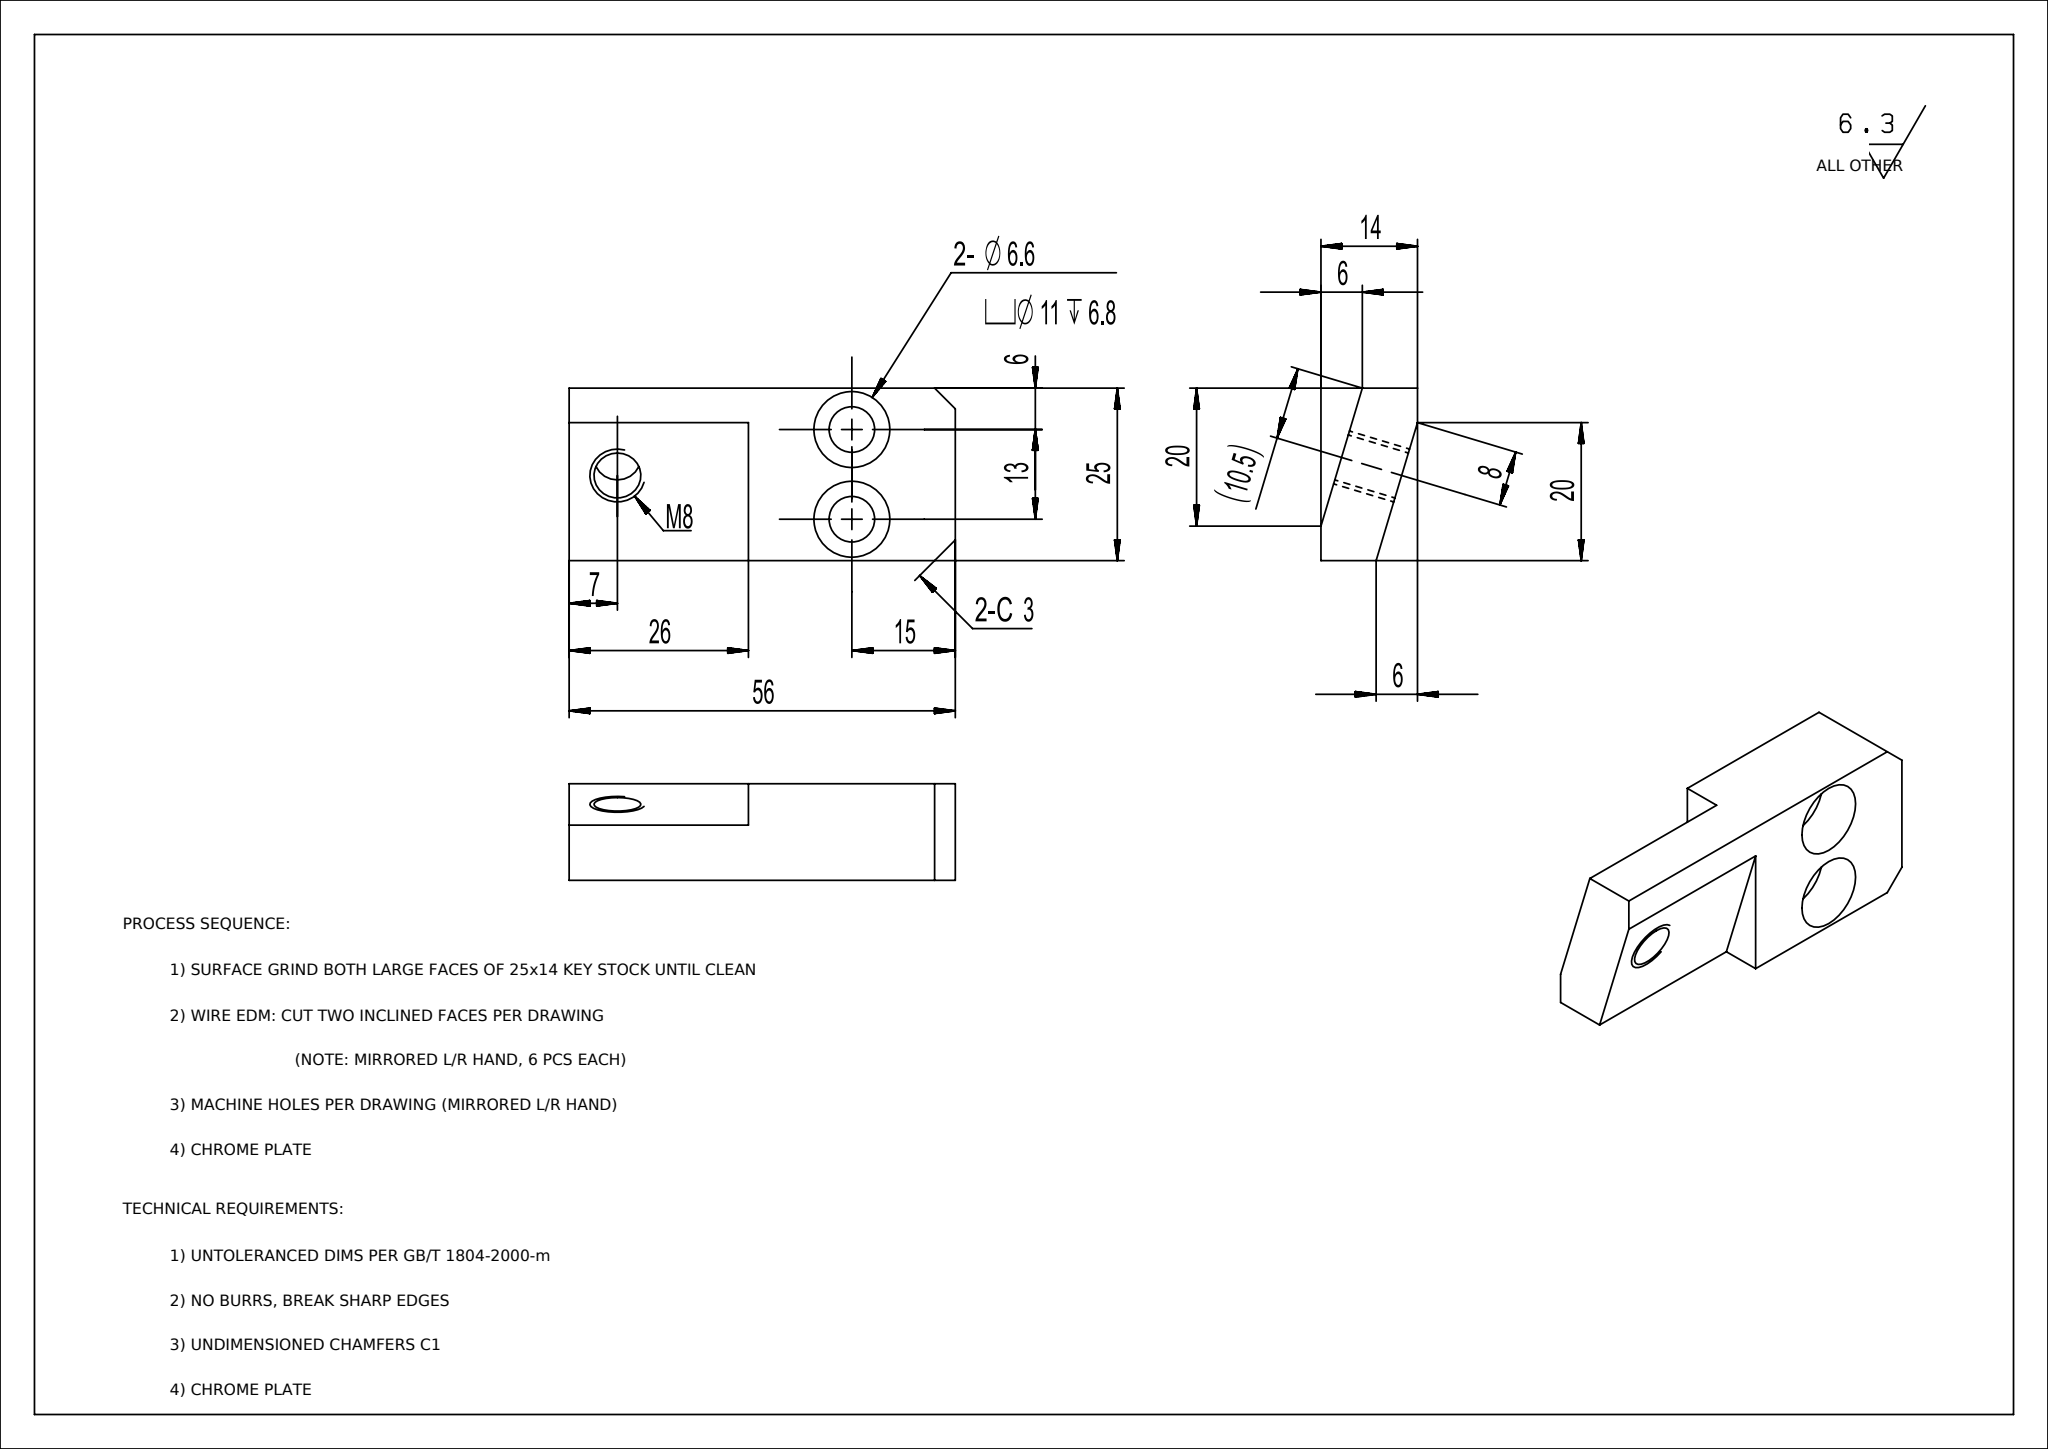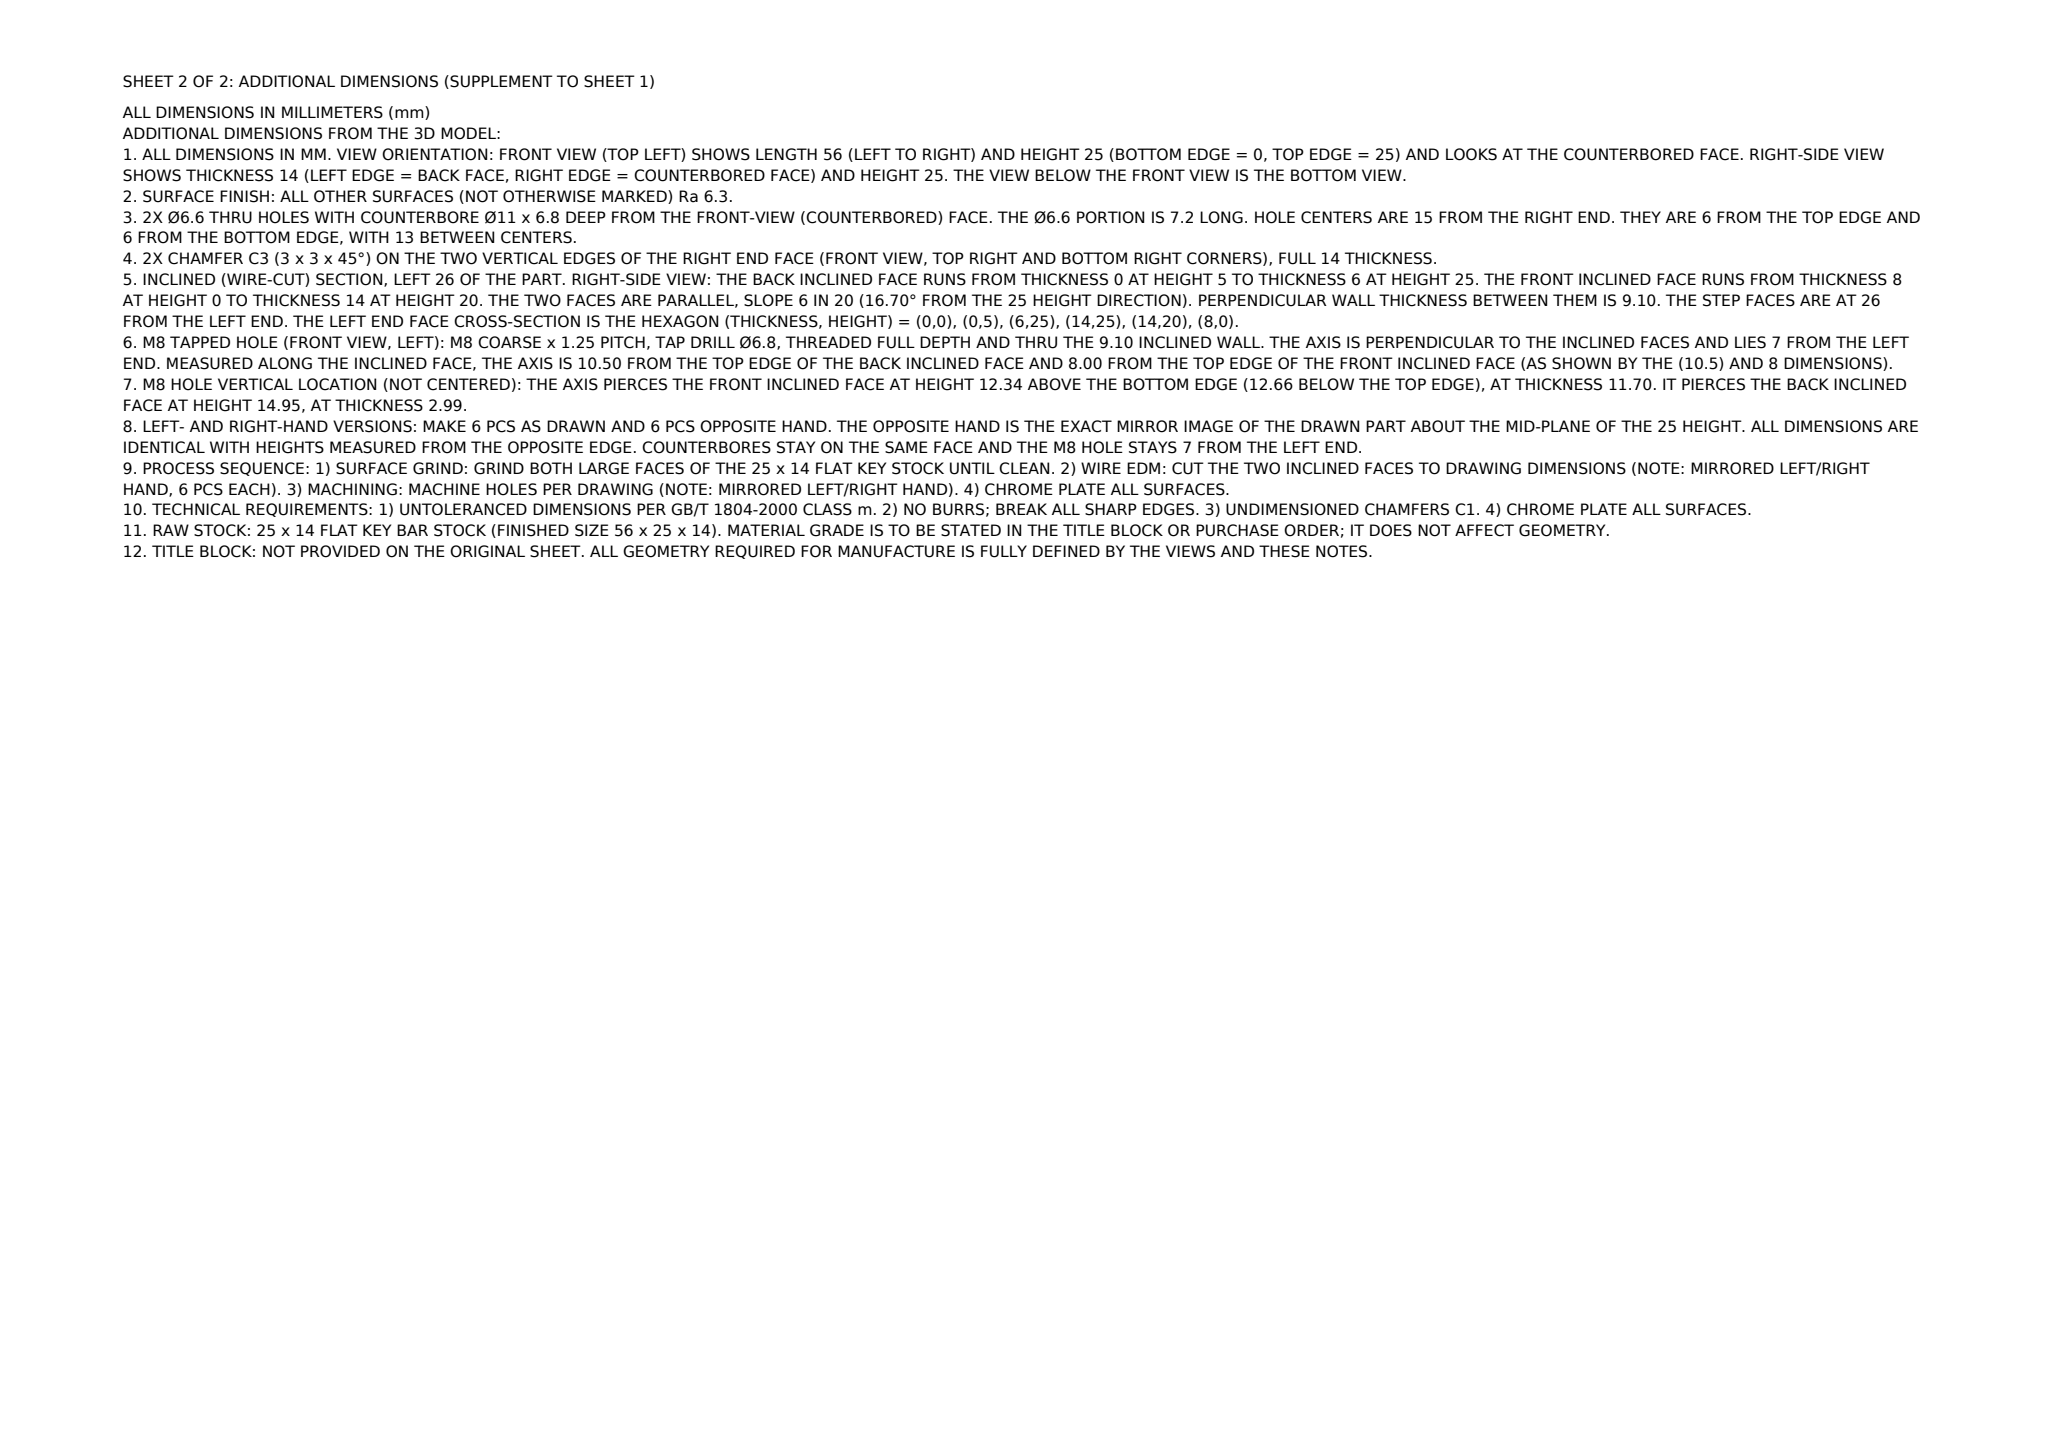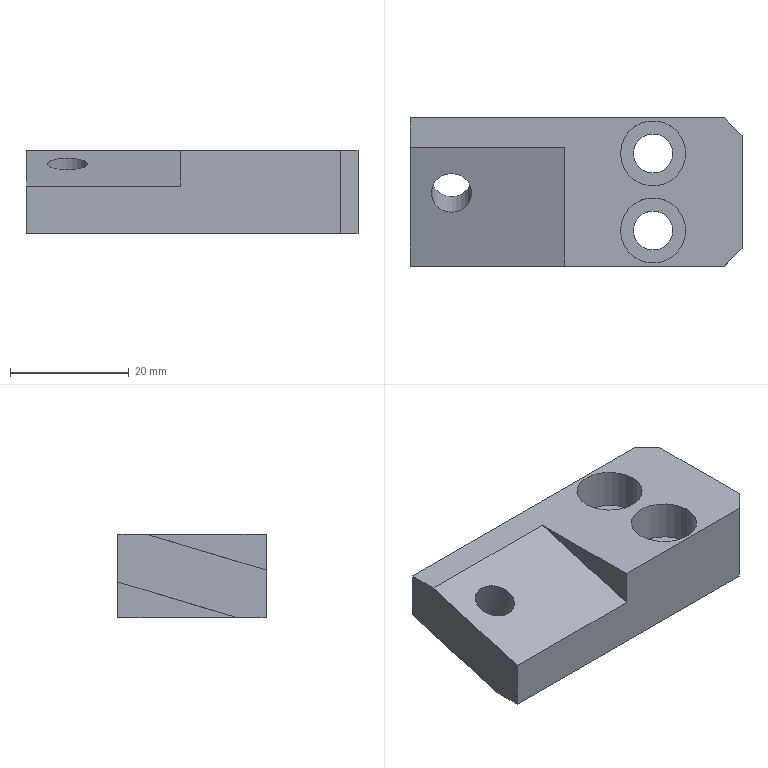Part | NX | mm | 1 solid | 19 faces | box 56 x 25 x 14 mm | volume 14238 mm3 | plane 14 | cylinder 5 | commonest cylinder face diameters 6.6 x2 11 x2 6.8 x1
STEP:
#1=CARTESIAN_POINT('',(0.,0.,0.));
#2=DIRECTION('',(0.,0.,1.));
#3=DIRECTION('',(1.,0.,0.));
#4=AXIS2_PLACEMENT_3D('',#1,#2,#3);
#5=(LENGTH_UNIT()NAMED_UNIT(*)SI_UNIT(.MILLI.,.METRE.));
#6=UNCERTAINTY_MEASURE_WITH_UNIT(LENGTH_MEASURE(0.00002),#5,'','');
#7=(NAMED_UNIT(*)PLANE_ANGLE_UNIT()SI_UNIT($,.RADIAN.));
#8=PLANE_ANGLE_MEASURE_WITH_UNIT(PLANE_ANGLE_MEASURE(0.01745),#7);
#9=DIMENSIONAL_EXPONENTS(0.,0.,0.,0.,0.,0.,0.);
#10=(CONVERSION_BASED_UNIT('',#8)NAMED_UNIT(#9)PLANE_ANGLE_UNIT());
#11=(NAMED_UNIT(*)SI_UNIT($,.STERADIAN.)SOLID_ANGLE_UNIT());
#12=(GEOMETRIC_REPRESENTATION_CONTEXT(3)GLOBAL_UNCERTAINTY_ASSIGNED_CONTEXT((#6))GLOBAL_UNIT_ASSIGNED_CONTEXT((#5,#10,#11))REPRESENTATION_CONTEXT('',''));
#13=SHAPE_REPRESENTATION('',(#4),#12);
#14=CARTESIAN_POINT('',(48.3,6.,0.));
#15=VERTEX_POINT('',#14);
#16=CARTESIAN_POINT('',(45.,6.,0.));
#17=DIRECTION('',(0.,0.,1.));
#18=DIRECTION('',(1.,0.,0.));
#19=AXIS2_PLACEMENT_3D('',#16,#17,#18);
#20=CIRCLE('',#19,3.3);
#21=EDGE_CURVE('',#15,#15,#20,.T.);
#22=ORIENTED_EDGE('',*,*,#21,.T.);
#23=EDGE_LOOP('',(#22));
#24=FACE_BOUND('',#23,.T.);
#25=CARTESIAN_POINT('',(48.3,19.,0.));
#26=VERTEX_POINT('',#25);
#27=CARTESIAN_POINT('',(45.,19.,0.));
#28=DIRECTION('',(0.,0.,1.));
#29=DIRECTION('',(1.,0.,0.));
#30=AXIS2_PLACEMENT_3D('',#27,#28,#29);
#31=CIRCLE('',#30,3.3);
#32=EDGE_CURVE('',#26,#26,#31,.T.);
#33=ORIENTED_EDGE('',*,*,#32,.T.);
#34=EDGE_LOOP('',(#33));
#35=FACE_BOUND('',#34,.T.);
#36=CARTESIAN_POINT('',(30.,25.,0.));
#37=VERTEX_POINT('',#36);
#38=CARTESIAN_POINT('',(30.,5.,0.));
#39=VERTEX_POINT('',#38);
#40=CARTESIAN_POINT('',(30.,25.,0.));
#41=DIRECTION('',(0.,-1.,0.));
#42=VECTOR('',#41,1.);
#43=LINE('',#40,#42);
#44=EDGE_CURVE('',#37,#39,#43,.T.);
#45=ORIENTED_EDGE('',*,*,#44,.F.);
#46=CARTESIAN_POINT('',(57.,25.,0.));
#47=VERTEX_POINT('',#46);
#48=CARTESIAN_POINT('',(60.,25.,0.));
#49=DIRECTION('',(-1.,0.,0.));
#50=VECTOR('',#49,1.);
#51=LINE('',#48,#50);
#52=EDGE_CURVE('',#47,#37,#51,.T.);
#53=ORIENTED_EDGE('',*,*,#52,.F.);
#54=CARTESIAN_POINT('',(60.,22.,0.));
#55=VERTEX_POINT('',#54);
#56=CARTESIAN_POINT('',(60.,22.,0.));
#57=DIRECTION('',(0.7071,-0.7071,0.));
#58=VECTOR('',#57,1.);
#59=LINE('',#56,#58);
#60=EDGE_CURVE('',#47,#55,#59,.T.);
#61=ORIENTED_EDGE('',*,*,#60,.T.);
#62=CARTESIAN_POINT('',(60.,3.,0.));
#63=VERTEX_POINT('',#62);
#64=CARTESIAN_POINT('',(60.,0.,0.));
#65=DIRECTION('',(0.,1.,0.));
#66=VECTOR('',#65,1.);
#67=LINE('',#64,#66);
#68=EDGE_CURVE('',#63,#55,#67,.T.);
#69=ORIENTED_EDGE('',*,*,#68,.F.);
#70=CARTESIAN_POINT('',(57.,0.,0.));
#71=VERTEX_POINT('',#70);
#72=CARTESIAN_POINT('',(60.,3.,0.));
#73=DIRECTION('',(-0.7071,-0.7071,0.));
#74=VECTOR('',#73,1.);
#75=LINE('',#72,#74);
#76=EDGE_CURVE('',#63,#71,#75,.T.);
#77=ORIENTED_EDGE('',*,*,#76,.T.);
#78=CARTESIAN_POINT('',(4.,0.,0.));
#79=VERTEX_POINT('',#78);
#80=CARTESIAN_POINT('',(60.,0.,0.));
#81=DIRECTION('',(-1.,0.,0.));
#82=VECTOR('',#81,1.);
#83=LINE('',#80,#82);
#84=EDGE_CURVE('',#71,#79,#83,.T.);
#85=ORIENTED_EDGE('',*,*,#84,.T.);
#86=CARTESIAN_POINT('',(4.,5.,0.));
#87=VERTEX_POINT('',#86);
#88=CARTESIAN_POINT('',(4.,0.,0.));
#89=DIRECTION('',(0.,1.,0.));
#90=VECTOR('',#89,1.);
#91=LINE('',#88,#90);
#92=EDGE_CURVE('',#79,#87,#91,.T.);
#93=ORIENTED_EDGE('',*,*,#92,.T.);
#94=CARTESIAN_POINT('',(30.,5.,0.));
#95=DIRECTION('',(-1.,0.,0.));
#96=VECTOR('',#95,1.);
#97=LINE('',#94,#96);
#98=EDGE_CURVE('',#39,#87,#97,.T.);
#99=ORIENTED_EDGE('',*,*,#98,.F.);
#100=EDGE_LOOP('',(#45,#53,#61,#69,#77,#85,#93,#99));
#101=FACE_BOUND('',#100,.T.);
#102=CARTESIAN_POINT('',(60.,0.,0.));
#103=DIRECTION('',(0.,0.,1.));
#104=DIRECTION('',(1.,0.,0.));
#105=AXIS2_PLACEMENT_3D('',#102,#103,#104);
#106=PLANE('',#105);
#107=ADVANCED_FACE('',(#24,#35,#101),#106,.F.);
#108=CARTESIAN_POINT('',(39.5,6.,14.));
#109=VERTEX_POINT('',#108);
#110=CARTESIAN_POINT('',(45.,6.,14.));
#111=DIRECTION('',(0.,0.,-1.));
#112=DIRECTION('',(-1.,0.,0.));
#113=AXIS2_PLACEMENT_3D('',#110,#111,#112);
#114=CIRCLE('',#113,5.5);
#115=EDGE_CURVE('',#109,#109,#114,.T.);
#116=ORIENTED_EDGE('',*,*,#115,.T.);
#117=EDGE_LOOP('',(#116));
#118=FACE_BOUND('',#117,.T.);
#119=CARTESIAN_POINT('',(39.5,19.,14.));
#120=VERTEX_POINT('',#119);
#121=CARTESIAN_POINT('',(45.,19.,14.));
#122=DIRECTION('',(0.,0.,-1.));
#123=DIRECTION('',(-1.,0.,0.));
#124=AXIS2_PLACEMENT_3D('',#121,#122,#123);
#125=CIRCLE('',#124,5.5);
#126=EDGE_CURVE('',#120,#120,#125,.T.);
#127=ORIENTED_EDGE('',*,*,#126,.T.);
#128=EDGE_LOOP('',(#127));
#129=FACE_BOUND('',#128,.T.);
#130=CARTESIAN_POINT('',(30.,0.,14.));
#131=VERTEX_POINT('',#130);
#132=CARTESIAN_POINT('',(30.,20.,14.));
#133=VERTEX_POINT('',#132);
#134=CARTESIAN_POINT('',(30.,0.,14.));
#135=DIRECTION('',(0.,1.,0.));
#136=VECTOR('',#135,1.);
#137=LINE('',#134,#136);
#138=EDGE_CURVE('',#131,#133,#137,.T.);
#139=ORIENTED_EDGE('',*,*,#138,.F.);
#140=CARTESIAN_POINT('',(57.,0.,14.));
#141=VERTEX_POINT('',#140);
#142=CARTESIAN_POINT('',(60.,0.,14.));
#143=DIRECTION('',(-1.,0.,0.));
#144=VECTOR('',#143,1.);
#145=LINE('',#142,#144);
#146=EDGE_CURVE('',#141,#131,#145,.T.);
#147=ORIENTED_EDGE('',*,*,#146,.F.);
#148=CARTESIAN_POINT('',(60.,3.,14.));
#149=VERTEX_POINT('',#148);
#150=CARTESIAN_POINT('',(60.,3.,14.));
#151=DIRECTION('',(0.7071,0.7071,0.));
#152=VECTOR('',#151,1.);
#153=LINE('',#150,#152);
#154=EDGE_CURVE('',#141,#149,#153,.T.);
#155=ORIENTED_EDGE('',*,*,#154,.T.);
#156=CARTESIAN_POINT('',(60.,22.,14.));
#157=VERTEX_POINT('',#156);
#158=CARTESIAN_POINT('',(60.,25.,14.));
#159=DIRECTION('',(0.,-1.,0.));
#160=VECTOR('',#159,1.);
#161=LINE('',#158,#160);
#162=EDGE_CURVE('',#157,#149,#161,.T.);
#163=ORIENTED_EDGE('',*,*,#162,.F.);
#164=CARTESIAN_POINT('',(57.,25.,14.));
#165=VERTEX_POINT('',#164);
#166=CARTESIAN_POINT('',(60.,22.,14.));
#167=DIRECTION('',(-0.7071,0.7071,0.));
#168=VECTOR('',#167,1.);
#169=LINE('',#166,#168);
#170=EDGE_CURVE('',#157,#165,#169,.T.);
#171=ORIENTED_EDGE('',*,*,#170,.T.);
#172=CARTESIAN_POINT('',(4.,25.,14.));
#173=VERTEX_POINT('',#172);
#174=CARTESIAN_POINT('',(60.,25.,14.));
#175=DIRECTION('',(-1.,0.,0.));
#176=VECTOR('',#175,1.);
#177=LINE('',#174,#176);
#178=EDGE_CURVE('',#165,#173,#177,.T.);
#179=ORIENTED_EDGE('',*,*,#178,.T.);
#180=CARTESIAN_POINT('',(4.,20.,14.));
#181=VERTEX_POINT('',#180);
#182=CARTESIAN_POINT('',(4.,25.,14.));
#183=DIRECTION('',(0.,-1.,0.));
#184=VECTOR('',#183,1.);
#185=LINE('',#182,#184);
#186=EDGE_CURVE('',#173,#181,#185,.T.);
#187=ORIENTED_EDGE('',*,*,#186,.T.);
#188=CARTESIAN_POINT('',(30.,20.,14.));
#189=DIRECTION('',(-1.,0.,0.));
#190=VECTOR('',#189,1.);
#191=LINE('',#188,#190);
#192=EDGE_CURVE('',#133,#181,#191,.T.);
#193=ORIENTED_EDGE('',*,*,#192,.F.);
#194=EDGE_LOOP('',(#139,#147,#155,#163,#171,#179,#187,#193));
#195=FACE_BOUND('',#194,.T.);
#196=CARTESIAN_POINT('',(60.,25.,14.));
#197=DIRECTION('',(0.,0.,-1.));
#198=DIRECTION('',(-1.,0.,0.));
#199=AXIS2_PLACEMENT_3D('',#196,#197,#198);
#200=PLANE('',#199);
#201=ADVANCED_FACE('',(#118,#129,#195),#200,.F.);
#202=CARTESIAN_POINT('',(4.,0.,8.));
#203=VERTEX_POINT('',#202);
#204=CARTESIAN_POINT('',(4.,20.,14.));
#205=DIRECTION('',(0.,-0.9578,-0.2873));
#206=VECTOR('',#205,1.);
#207=LINE('',#204,#206);
#208=EDGE_CURVE('',#181,#203,#207,.T.);
#209=ORIENTED_EDGE('',*,*,#208,.F.);
#210=ORIENTED_EDGE('',*,*,#186,.F.);
#211=CARTESIAN_POINT('',(4.,25.,6.));
#212=VERTEX_POINT('',#211);
#213=CARTESIAN_POINT('',(4.,25.,0.));
#214=DIRECTION('',(0.,-0.,1.));
#215=VECTOR('',#214,1.);
#216=LINE('',#213,#215);
#217=EDGE_CURVE('',#212,#173,#216,.T.);
#218=ORIENTED_EDGE('',*,*,#217,.F.);
#219=CARTESIAN_POINT('',(4.,5.,0.));
#220=DIRECTION('',(0.,0.9578,0.2873));
#221=VECTOR('',#220,1.);
#222=LINE('',#219,#221);
#223=EDGE_CURVE('',#87,#212,#222,.T.);
#224=ORIENTED_EDGE('',*,*,#223,.F.);
#225=ORIENTED_EDGE('',*,*,#92,.F.);
#226=CARTESIAN_POINT('',(4.,0.,14.));
#227=DIRECTION('',(0.,0.,-1.));
#228=VECTOR('',#227,1.);
#229=LINE('',#226,#228);
#230=EDGE_CURVE('',#203,#79,#229,.T.);
#231=ORIENTED_EDGE('',*,*,#230,.F.);
#232=EDGE_LOOP('',(#209,#210,#218,#224,#225,#231));
#233=FACE_OUTER_BOUND('',#232,.T.);
#234=CARTESIAN_POINT('',(4.,0.,0.));
#235=DIRECTION('',(1.,0.,0.));
#236=DIRECTION('',(0.,0.,-1.));
#237=AXIS2_PLACEMENT_3D('',#234,#235,#236);
#238=PLANE('',#237);
#239=ADVANCED_FACE('',(#233),#238,.F.);
#240=CARTESIAN_POINT('',(30.,0.,8.));
#241=VERTEX_POINT('',#240);
#242=CARTESIAN_POINT('',(30.,0.,8.));
#243=DIRECTION('',(0.,0.,1.));
#244=VECTOR('',#243,1.);
#245=LINE('',#242,#244);
#246=EDGE_CURVE('',#241,#131,#245,.T.);
#247=ORIENTED_EDGE('',*,*,#246,.F.);
#248=CARTESIAN_POINT('',(30.,0.,8.));
#249=DIRECTION('',(-1.,0.,0.));
#250=VECTOR('',#249,1.);
#251=LINE('',#248,#250);
#252=EDGE_CURVE('',#241,#203,#251,.T.);
#253=ORIENTED_EDGE('',*,*,#252,.T.);
#254=ORIENTED_EDGE('',*,*,#230,.T.);
#255=ORIENTED_EDGE('',*,*,#84,.F.);
#256=CARTESIAN_POINT('',(57.,0.,14.));
#257=DIRECTION('',(0.,0.,1.));
#258=VECTOR('',#257,1.);
#259=LINE('',#256,#258);
#260=EDGE_CURVE('',#71,#141,#259,.T.);
#261=ORIENTED_EDGE('',*,*,#260,.T.);
#262=ORIENTED_EDGE('',*,*,#146,.T.);
#263=EDGE_LOOP('',(#247,#253,#254,#255,#261,#262));
#264=FACE_OUTER_BOUND('',#263,.T.);
#265=CARTESIAN_POINT('',(60.,0.,14.));
#266=DIRECTION('',(0.,1.,0.));
#267=DIRECTION('',(0.,0.,1.));
#268=AXIS2_PLACEMENT_3D('',#265,#266,#267);
#269=PLANE('',#268);
#270=ADVANCED_FACE('',(#264),#269,.F.);
#271=CARTESIAN_POINT('',(30.,25.,6.));
#272=VERTEX_POINT('',#271);
#273=CARTESIAN_POINT('',(30.,25.,6.));
#274=DIRECTION('',(0.,0.,-1.));
#275=VECTOR('',#274,1.);
#276=LINE('',#273,#275);
#277=EDGE_CURVE('',#272,#37,#276,.T.);
#278=ORIENTED_EDGE('',*,*,#277,.F.);
#279=CARTESIAN_POINT('',(30.,25.,6.));
#280=DIRECTION('',(-1.,0.,0.));
#281=VECTOR('',#280,1.);
#282=LINE('',#279,#281);
#283=EDGE_CURVE('',#272,#212,#282,.T.);
#284=ORIENTED_EDGE('',*,*,#283,.T.);
#285=ORIENTED_EDGE('',*,*,#217,.T.);
#286=ORIENTED_EDGE('',*,*,#178,.F.);
#287=CARTESIAN_POINT('',(57.,25.,0.));
#288=DIRECTION('',(0.,0.,-1.));
#289=VECTOR('',#288,1.);
#290=LINE('',#287,#289);
#291=EDGE_CURVE('',#165,#47,#290,.T.);
#292=ORIENTED_EDGE('',*,*,#291,.T.);
#293=ORIENTED_EDGE('',*,*,#52,.T.);
#294=EDGE_LOOP('',(#278,#284,#285,#286,#292,#293));
#295=FACE_OUTER_BOUND('',#294,.T.);
#296=CARTESIAN_POINT('',(60.,25.,0.));
#297=DIRECTION('',(0.,-1.,-0.));
#298=DIRECTION('',(0.,0.,-1.));
#299=AXIS2_PLACEMENT_3D('',#296,#297,#298);
#300=PLANE('',#299);
#301=ADVANCED_FACE('',(#295),#300,.F.);
#302=ORIENTED_EDGE('',*,*,#68,.T.);
#303=CARTESIAN_POINT('',(60.,22.,14.));
#304=DIRECTION('',(0.,-0.,1.));
#305=VECTOR('',#304,1.);
#306=LINE('',#303,#305);
#307=EDGE_CURVE('',#55,#157,#306,.T.);
#308=ORIENTED_EDGE('',*,*,#307,.T.);
#309=ORIENTED_EDGE('',*,*,#162,.T.);
#310=CARTESIAN_POINT('',(60.,3.,0.));
#311=DIRECTION('',(0.,0.,-1.));
#312=VECTOR('',#311,1.);
#313=LINE('',#310,#312);
#314=EDGE_CURVE('',#149,#63,#313,.T.);
#315=ORIENTED_EDGE('',*,*,#314,.T.);
#316=EDGE_LOOP('',(#302,#308,#309,#315));
#317=FACE_OUTER_BOUND('',#316,.T.);
#318=CARTESIAN_POINT('',(60.,0.,0.));
#319=DIRECTION('',(1.,0.,0.));
#320=DIRECTION('',(0.,0.,-1.));
#321=AXIS2_PLACEMENT_3D('',#318,#319,#320);
#322=PLANE('',#321);
#323=ADVANCED_FACE('',(#317),#322,.T.);
#324=CARTESIAN_POINT('',(41.7,6.,7.2));
#325=VERTEX_POINT('',#324);
#326=CARTESIAN_POINT('',(45.,6.,7.2));
#327=DIRECTION('',(0.,0.,1.));
#328=DIRECTION('',(-1.,0.,0.));
#329=AXIS2_PLACEMENT_3D('',#326,#327,#328);
#330=CIRCLE('',#329,3.3);
#331=EDGE_CURVE('',#325,#325,#330,.T.);
#332=ORIENTED_EDGE('',*,*,#331,.T.);
#333=EDGE_LOOP('',(#332));
#334=FACE_BOUND('',#333,.T.);
#335=ORIENTED_EDGE('',*,*,#21,.F.);
#336=EDGE_LOOP('',(#335));
#337=FACE_BOUND('',#336,.T.);
#338=CARTESIAN_POINT('',(45.,6.,-36.));
#339=DIRECTION('',(0.,0.,-1.));
#340=DIRECTION('',(-1.,0.,0.));
#341=AXIS2_PLACEMENT_3D('',#338,#339,#340);
#342=CYLINDRICAL_SURFACE('',#341,3.3);
#343=ADVANCED_FACE('',(#334,#337),#342,.F.);
#344=ORIENTED_EDGE('',*,*,#331,.F.);
#345=EDGE_LOOP('',(#344));
#346=FACE_BOUND('',#345,.T.);
#347=CARTESIAN_POINT('',(39.5,6.,7.2));
#348=VERTEX_POINT('',#347);
#349=CARTESIAN_POINT('',(45.,6.,7.2));
#350=DIRECTION('',(0.,0.,1.));
#351=DIRECTION('',(-1.,0.,0.));
#352=AXIS2_PLACEMENT_3D('',#349,#350,#351);
#353=CIRCLE('',#352,5.5);
#354=EDGE_CURVE('',#348,#348,#353,.T.);
#355=ORIENTED_EDGE('',*,*,#354,.T.);
#356=EDGE_LOOP('',(#355));
#357=FACE_BOUND('',#356,.T.);
#358=CARTESIAN_POINT('',(45.,6.,7.2));
#359=DIRECTION('',(0.,0.,-1.));
#360=DIRECTION('',(-1.,0.,0.));
#361=AXIS2_PLACEMENT_3D('',#358,#359,#360);
#362=PLANE('',#361);
#363=ADVANCED_FACE('',(#346,#357),#362,.F.);
#364=ORIENTED_EDGE('',*,*,#354,.F.);
#365=EDGE_LOOP('',(#364));
#366=FACE_BOUND('',#365,.T.);
#367=ORIENTED_EDGE('',*,*,#115,.F.);
#368=EDGE_LOOP('',(#367));
#369=FACE_BOUND('',#368,.T.);
#370=CARTESIAN_POINT('',(45.,6.,14.));
#371=DIRECTION('',(0.,0.,-1.));
#372=DIRECTION('',(-1.,0.,0.));
#373=AXIS2_PLACEMENT_3D('',#370,#371,#372);
#374=CYLINDRICAL_SURFACE('',#373,5.5);
#375=ADVANCED_FACE('',(#366,#369),#374,.F.);
#376=CARTESIAN_POINT('',(41.7,19.,7.2));
#377=VERTEX_POINT('',#376);
#378=CARTESIAN_POINT('',(45.,19.,7.2));
#379=DIRECTION('',(0.,0.,1.));
#380=DIRECTION('',(-1.,0.,0.));
#381=AXIS2_PLACEMENT_3D('',#378,#379,#380);
#382=CIRCLE('',#381,3.3);
#383=EDGE_CURVE('',#377,#377,#382,.T.);
#384=ORIENTED_EDGE('',*,*,#383,.T.);
#385=EDGE_LOOP('',(#384));
#386=FACE_BOUND('',#385,.T.);
#387=ORIENTED_EDGE('',*,*,#32,.F.);
#388=EDGE_LOOP('',(#387));
#389=FACE_BOUND('',#388,.T.);
#390=CARTESIAN_POINT('',(45.,19.,-36.));
#391=DIRECTION('',(0.,0.,-1.));
#392=DIRECTION('',(-1.,0.,0.));
#393=AXIS2_PLACEMENT_3D('',#390,#391,#392);
#394=CYLINDRICAL_SURFACE('',#393,3.3);
#395=ADVANCED_FACE('',(#386,#389),#394,.F.);
#396=ORIENTED_EDGE('',*,*,#383,.F.);
#397=EDGE_LOOP('',(#396));
#398=FACE_BOUND('',#397,.T.);
#399=CARTESIAN_POINT('',(39.5,19.,7.2));
#400=VERTEX_POINT('',#399);
#401=CARTESIAN_POINT('',(45.,19.,7.2));
#402=DIRECTION('',(0.,0.,1.));
#403=DIRECTION('',(-1.,0.,0.));
#404=AXIS2_PLACEMENT_3D('',#401,#402,#403);
#405=CIRCLE('',#404,5.5);
#406=EDGE_CURVE('',#400,#400,#405,.T.);
#407=ORIENTED_EDGE('',*,*,#406,.T.);
#408=EDGE_LOOP('',(#407));
#409=FACE_BOUND('',#408,.T.);
#410=CARTESIAN_POINT('',(45.,19.,7.2));
#411=DIRECTION('',(0.,0.,-1.));
#412=DIRECTION('',(-1.,0.,0.));
#413=AXIS2_PLACEMENT_3D('',#410,#411,#412);
#414=PLANE('',#413);
#415=ADVANCED_FACE('',(#398,#409),#414,.F.);
#416=ORIENTED_EDGE('',*,*,#406,.F.);
#417=EDGE_LOOP('',(#416));
#418=FACE_BOUND('',#417,.T.);
#419=ORIENTED_EDGE('',*,*,#126,.F.);
#420=EDGE_LOOP('',(#419));
#421=FACE_BOUND('',#420,.T.);
#422=CARTESIAN_POINT('',(45.,19.,14.));
#423=DIRECTION('',(0.,0.,-1.));
#424=DIRECTION('',(-1.,0.,0.));
#425=AXIS2_PLACEMENT_3D('',#422,#423,#424);
#426=CYLINDRICAL_SURFACE('',#425,5.5);
#427=ADVANCED_FACE('',(#418,#421),#426,.F.);
#428=ORIENTED_EDGE('',*,*,#60,.F.);
#429=ORIENTED_EDGE('',*,*,#291,.F.);
#430=ORIENTED_EDGE('',*,*,#170,.F.);
#431=ORIENTED_EDGE('',*,*,#307,.F.);
#432=EDGE_LOOP('',(#428,#429,#430,#431));
#433=FACE_OUTER_BOUND('',#432,.T.);
#434=CARTESIAN_POINT('',(60.,22.,0.));
#435=DIRECTION('',(0.7071,0.7071,0.));
#436=DIRECTION('',(0.,0.,-1.));
#437=AXIS2_PLACEMENT_3D('',#434,#435,#436);
#438=PLANE('',#437);
#439=ADVANCED_FACE('',(#433),#438,.T.);
#440=ORIENTED_EDGE('',*,*,#154,.F.);
#441=ORIENTED_EDGE('',*,*,#260,.F.);
#442=ORIENTED_EDGE('',*,*,#76,.F.);
#443=ORIENTED_EDGE('',*,*,#314,.F.);
#444=EDGE_LOOP('',(#440,#441,#442,#443));
#445=FACE_OUTER_BOUND('',#444,.T.);
#446=CARTESIAN_POINT('',(60.,3.,0.));
#447=DIRECTION('',(0.7071,-0.7071,0.));
#448=DIRECTION('',(0.,0.,1.));
#449=AXIS2_PLACEMENT_3D('',#446,#447,#448);
#450=PLANE('',#449);
#451=ADVANCED_FACE('',(#445),#450,.T.);
#452=CARTESIAN_POINT('',(11.,11.695,2.009));
#453=VERTEX_POINT('',#452);
#454=CARTESIAN_POINT('',(11.,14.952,2.986));
#455=DIRECTION('',(0.,-0.2873,0.9578));
#456=DIRECTION('',(0.,-0.9578,-0.2873));
#457=AXIS2_PLACEMENT_3D('',#454,#455,#456);
#458=CIRCLE('',#457,3.4);
#459=EDGE_CURVE('',#453,#453,#458,.T.);
#460=ORIENTED_EDGE('',*,*,#459,.T.);
#461=EDGE_LOOP('',(#460));
#462=FACE_BOUND('',#461,.T.);
#463=ORIENTED_EDGE('',*,*,#223,.T.);
#464=ORIENTED_EDGE('',*,*,#283,.F.);
#465=CARTESIAN_POINT('',(30.,5.,0.));
#466=DIRECTION('',(0.,-0.9578,-0.2873));
#467=VECTOR('',#466,1.);
#468=LINE('',#465,#467);
#469=EDGE_CURVE('',#272,#39,#468,.T.);
#470=ORIENTED_EDGE('',*,*,#469,.T.);
#471=ORIENTED_EDGE('',*,*,#98,.T.);
#472=EDGE_LOOP('',(#463,#464,#470,#471));
#473=FACE_BOUND('',#472,.T.);
#474=CARTESIAN_POINT('',(30.,5.,0.));
#475=DIRECTION('',(0.,-0.2873,0.9578));
#476=DIRECTION('',(0.,-0.9578,-0.2873));
#477=AXIS2_PLACEMENT_3D('',#474,#475,#476);
#478=PLANE('',#477);
#479=ADVANCED_FACE('',(#462,#473),#478,.F.);
#480=ORIENTED_EDGE('',*,*,#44,.T.);
#481=ORIENTED_EDGE('',*,*,#469,.F.);
#482=ORIENTED_EDGE('',*,*,#277,.T.);
#483=EDGE_LOOP('',(#480,#481,#482));
#484=FACE_OUTER_BOUND('',#483,.T.);
#485=CARTESIAN_POINT('',(30.,0.,0.));
#486=DIRECTION('',(1.,0.,0.));
#487=DIRECTION('',(0.,0.,-1.));
#488=AXIS2_PLACEMENT_3D('',#485,#486,#487);
#489=PLANE('',#488);
#490=ADVANCED_FACE('',(#484),#489,.F.);
#491=CARTESIAN_POINT('',(11.,15.594,12.678));
#492=VERTEX_POINT('',#491);
#493=CARTESIAN_POINT('',(11.,12.337,11.701));
#494=DIRECTION('',(0.,0.2873,-0.9578));
#495=DIRECTION('',(0.,0.9578,0.2873));
#496=AXIS2_PLACEMENT_3D('',#493,#494,#495);
#497=CIRCLE('',#496,3.4);
#498=EDGE_CURVE('',#492,#492,#497,.T.);
#499=ORIENTED_EDGE('',*,*,#498,.T.);
#500=EDGE_LOOP('',(#499));
#501=FACE_BOUND('',#500,.T.);
#502=ORIENTED_EDGE('',*,*,#208,.T.);
#503=ORIENTED_EDGE('',*,*,#252,.F.);
#504=CARTESIAN_POINT('',(30.,20.,14.));
#505=DIRECTION('',(0.,0.9578,0.2873));
#506=VECTOR('',#505,1.);
#507=LINE('',#504,#506);
#508=EDGE_CURVE('',#241,#133,#507,.T.);
#509=ORIENTED_EDGE('',*,*,#508,.T.);
#510=ORIENTED_EDGE('',*,*,#192,.T.);
#511=EDGE_LOOP('',(#502,#503,#509,#510));
#512=FACE_BOUND('',#511,.T.);
#513=CARTESIAN_POINT('',(30.,20.,14.));
#514=DIRECTION('',(0.,0.2873,-0.9578));
#515=DIRECTION('',(0.,0.9578,0.2873));
#516=AXIS2_PLACEMENT_3D('',#513,#514,#515);
#517=PLANE('',#516);
#518=ADVANCED_FACE('',(#501,#512),#517,.F.);
#519=ORIENTED_EDGE('',*,*,#246,.T.);
#520=ORIENTED_EDGE('',*,*,#138,.T.);
#521=ORIENTED_EDGE('',*,*,#508,.F.);
#522=EDGE_LOOP('',(#519,#520,#521));
#523=FACE_OUTER_BOUND('',#522,.T.);
#524=CARTESIAN_POINT('',(30.,0.,0.));
#525=DIRECTION('',(-1.,0.,0.));
#526=DIRECTION('',(0.,0.,1.));
#527=AXIS2_PLACEMENT_3D('',#524,#525,#526);
#528=PLANE('',#527);
#529=ADVANCED_FACE('',(#523),#528,.T.);
#530=ORIENTED_EDGE('',*,*,#498,.F.);
#531=EDGE_LOOP('',(#530));
#532=FACE_BOUND('',#531,.T.);
#533=ORIENTED_EDGE('',*,*,#459,.F.);
#534=EDGE_LOOP('',(#533));
#535=FACE_BOUND('',#534,.T.);
#536=CARTESIAN_POINT('',(11.,12.337,11.701));
#537=DIRECTION('',(0.,0.2873,-0.9578));
#538=DIRECTION('',(0.,0.9578,0.2873));
#539=AXIS2_PLACEMENT_3D('',#536,#537,#538);
#540=CYLINDRICAL_SURFACE('',#539,3.4);
#541=ADVANCED_FACE('',(#532,#535),#540,.F.);
#542=CLOSED_SHELL('',(#107,#201,#239,#270,#301,#323,#343,#363,#375,#395,#415,#427,#439,#451,#479,#490,#518,#529,#541));
#543=MANIFOLD_SOLID_BREP('',#542);
#544=ADVANCED_BREP_SHAPE_REPRESENTATION('',(#543),#12);
#545=SHAPE_REPRESENTATION_RELATIONSHIP('','',#13,#544);
#546=PRESENTATION_LAYER_ASSIGNMENT('','',(#543));
#547=COLOUR_RGB('',0.8745,0.8745,0.8745);
#548=FILL_AREA_STYLE_COLOUR('',#547);
#549=FILL_AREA_STYLE('',(#548));
#550=SURFACE_STYLE_FILL_AREA(#549);
#551=SURFACE_SIDE_STYLE('',(#550));
#552=SURFACE_STYLE_USAGE(.BOTH.,#551);
#553=PRESENTATION_STYLE_ASSIGNMENT((#552));
#554=STYLED_ITEM('',(#553),#543);
#555=MECHANICAL_DESIGN_GEOMETRIC_PRESENTATION_REPRESENTATION('',(#554),#12);